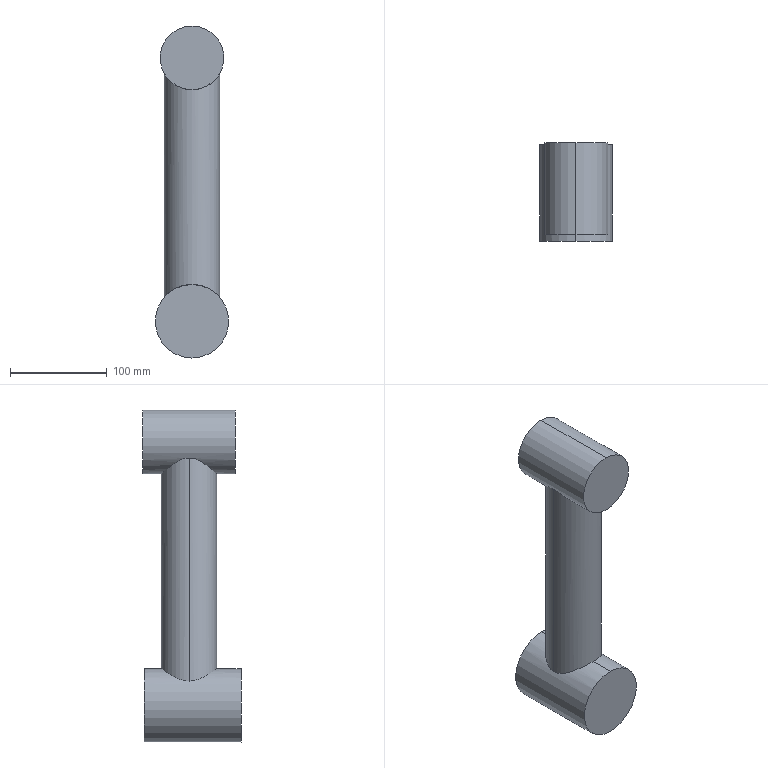Component | SolidWorks | RehabilitationChair-18-8-2 | 1 solid | 12 faces | box 75.75 x 101.12 x 342.27 mm | volume 1304986 mm3 | cylinder 6 | plane 6 | commonest cylinder face diameters 75.746 x2 65.746 x2 57.165 x2
STEP:
#1=COLOUR_RGB('',0.7922,0.8196,0.9333);
#2=FILL_AREA_STYLE_COLOUR('',#1);
#3=FILL_AREA_STYLE('',(#2));
#4=SURFACE_STYLE_FILL_AREA(#3);
#5=SURFACE_SIDE_STYLE('',(#4));
#6=SURFACE_STYLE_USAGE(.BOTH.,#5);
#7=PRESENTATION_STYLE_ASSIGNMENT((#6));
#8=CARTESIAN_POINT('',(-6.121,12.801,6.194));
#9=VERTEX_POINT('',#8);
#10=CARTESIAN_POINT('',(-6.121,12.801,3.212));
#11=VERTEX_POINT('',#10);
#12=CARTESIAN_POINT('',(-6.121,12.801,4.703));
#13=DIRECTION('',(-0.00000124,-1.,-0.));
#14=DIRECTION('',(-0.00000052,0.,1.));
#15=AXIS2_PLACEMENT_3D('',#12,#13,#14);
#16=CIRCLE('',#15,1.491);
#17=EDGE_CURVE('',#9,#11,#16,.T.);
#18=ORIENTED_EDGE('',*,*,#17,.F.);
#19=CARTESIAN_POINT('',(-6.121,13.786,6.194));
#20=VERTEX_POINT('',#19);
#21=CARTESIAN_POINT('',(-6.121,12.801,6.194));
#22=DIRECTION('',(0.00000124,1.,0.));
#23=VECTOR('',#22,39.37);
#24=LINE('',#21,#23);
#25=EDGE_CURVE('',#9,#20,#24,.T.);
#26=ORIENTED_EDGE('',*,*,#25,.T.);
#27=CARTESIAN_POINT('',(-7.246,14.911,5.682));
#28=VERTEX_POINT('',#27);
#29=CARTESIAN_POINT('',(-7.246,14.911,5.682));
#30=CARTESIAN_POINT('',(-7.246,14.833,5.682));
#31=CARTESIAN_POINT('',(-7.238,14.757,5.691));
#32=CARTESIAN_POINT('',(-7.219,14.664,5.712));
#33=CARTESIAN_POINT('',(-7.215,14.646,5.717));
#34=CARTESIAN_POINT('',(-7.205,14.61,5.727));
#35=CARTESIAN_POINT('',(-7.2,14.592,5.732));
#36=CARTESIAN_POINT('',(-7.183,14.539,5.749));
#37=CARTESIAN_POINT('',(-7.171,14.504,5.762));
#38=CARTESIAN_POINT('',(-7.128,14.405,5.803));
#39=CARTESIAN_POINT('',(-7.094,14.342,5.834));
#40=CARTESIAN_POINT('',(-7.015,14.224,5.897));
#41=CARTESIAN_POINT('',(-6.971,14.17,5.93));
#42=CARTESIAN_POINT('',(-6.896,14.095,5.977));
#43=CARTESIAN_POINT('',(-6.87,14.071,5.993));
#44=CARTESIAN_POINT('',(-6.829,14.037,6.015));
#45=CARTESIAN_POINT('',(-6.815,14.025,6.023));
#46=CARTESIAN_POINT('',(-6.787,14.004,6.038));
#47=CARTESIAN_POINT('',(-6.772,13.993,6.045));
#48=CARTESIAN_POINT('',(-6.698,13.942,6.08));
#49=CARTESIAN_POINT('',(-6.634,13.907,6.105));
#50=CARTESIAN_POINT('',(-6.531,13.863,6.137));
#51=CARTESIAN_POINT('',(-6.496,13.849,6.147));
#52=CARTESIAN_POINT('',(-6.424,13.827,6.164));
#53=CARTESIAN_POINT('',(-6.387,13.817,6.171));
#54=CARTESIAN_POINT('',(-6.313,13.802,6.182));
#55=CARTESIAN_POINT('',(-6.275,13.796,6.187));
#56=CARTESIAN_POINT('',(-6.218,13.79,6.191));
#57=CARTESIAN_POINT('',(-6.199,13.788,6.192));
#58=CARTESIAN_POINT('',(-6.16,13.786,6.194));
#59=CARTESIAN_POINT('',(-6.14,13.786,6.194));
#60=CARTESIAN_POINT('',(-6.121,13.786,6.194));
#61=B_SPLINE_CURVE_WITH_KNOTS('',3,(#29,#30,#31,#32,#33,#34,#35,#36,#37,#38,#39,#40,#41,#42,#43,#44,#45,#46,#47,#48,#49,#50,#51,#52,#53,#54,#55,#56,#57,#58,#59,#60),.UNSPECIFIED.,.F.,.F.,(4,2,2,2,2,2,2,2,2,2,2,2,2,2,2,4),(0.,0.005855,0.007319,0.008782,0.01171,0.01756,0.02342,0.02635,0.02781,0.02927,0.03513,0.03806,0.04098,0.04391,0.04538,0.04684),.UNSPECIFIED.);
#62=EDGE_CURVE('',#28,#20,#61,.T.);
#63=ORIENTED_EDGE('',*,*,#62,.F.);
#64=CARTESIAN_POINT('',(-6.121,16.036,6.194));
#65=VERTEX_POINT('',#64);
#66=CARTESIAN_POINT('',(-6.121,16.036,6.194));
#67=CARTESIAN_POINT('',(-6.199,16.036,6.194));
#68=CARTESIAN_POINT('',(-6.275,16.028,6.188));
#69=CARTESIAN_POINT('',(-6.387,16.005,6.171));
#70=CARTESIAN_POINT('',(-6.424,15.995,6.164));
#71=CARTESIAN_POINT('',(-6.496,15.972,6.147));
#72=CARTESIAN_POINT('',(-6.531,15.959,6.137));
#73=CARTESIAN_POINT('',(-6.599,15.93,6.116));
#74=CARTESIAN_POINT('',(-6.632,15.914,6.104));
#75=CARTESIAN_POINT('',(-6.681,15.887,6.085));
#76=CARTESIAN_POINT('',(-6.697,15.878,6.079));
#77=CARTESIAN_POINT('',(-6.728,15.859,6.065));
#78=CARTESIAN_POINT('',(-6.743,15.849,6.059));
#79=CARTESIAN_POINT('',(-6.817,15.798,6.023));
#80=CARTESIAN_POINT('',(-6.871,15.753,5.993));
#81=CARTESIAN_POINT('',(-6.933,15.69,5.953));
#82=CARTESIAN_POINT('',(-6.946,15.677,5.945));
#83=CARTESIAN_POINT('',(-6.969,15.65,5.929));
#84=CARTESIAN_POINT('',(-6.981,15.637,5.921));
#85=CARTESIAN_POINT('',(-7.014,15.596,5.897));
#86=CARTESIAN_POINT('',(-7.035,15.568,5.881));
#87=CARTESIAN_POINT('',(-7.074,15.51,5.85));
#88=CARTESIAN_POINT('',(-7.092,15.48,5.835));
#89=CARTESIAN_POINT('',(-7.118,15.433,5.812));
#90=CARTESIAN_POINT('',(-7.126,15.417,5.805));
#91=CARTESIAN_POINT('',(-7.142,15.385,5.79));
#92=CARTESIAN_POINT('',(-7.149,15.368,5.783));
#93=CARTESIAN_POINT('',(-7.185,15.285,5.749));
#94=CARTESIAN_POINT('',(-7.207,15.215,5.725));
#95=CARTESIAN_POINT('',(-7.23,15.104,5.7));
#96=CARTESIAN_POINT('',(-7.236,15.065,5.693));
#97=CARTESIAN_POINT('',(-7.244,14.989,5.684));
#98=CARTESIAN_POINT('',(-7.246,14.95,5.682));
#99=CARTESIAN_POINT('',(-7.246,14.911,5.682));
#100=B_SPLINE_CURVE_WITH_KNOTS('',3,(#66,#67,#68,#69,#70,#71,#72,#73,#74,#75,#76,#77,#78,#79,#80,#81,#82,#83,#84,#85,#86,#87,#88,#89,#90,#91,#92,#93,#94,#95,#96,#97,#98,#99),.UNSPECIFIED.,.F.,.F.,(4,2,2,2,2,2,2,2,2,2,2,2,2,2,2,2,4),(0.1403,0.1462,0.1491,0.152,0.1549,0.1564,0.1578,0.1637,0.1651,0.1666,0.1695,0.1724,0.1739,0.1753,0.1811,0.1841,0.187),.UNSPECIFIED.);
#101=EDGE_CURVE('',#65,#28,#100,.T.);
#102=ORIENTED_EDGE('',*,*,#101,.F.);
#103=CARTESIAN_POINT('',(-6.121,16.738,6.194));
#104=VERTEX_POINT('',#103);
#105=CARTESIAN_POINT('',(-6.121,12.801,6.194));
#106=DIRECTION('',(0.00000124,1.,0.));
#107=VECTOR('',#106,39.37);
#108=LINE('',#105,#107);
#109=EDGE_CURVE('',#65,#104,#108,.T.);
#110=ORIENTED_EDGE('',*,*,#109,.T.);
#111=CARTESIAN_POINT('',(-6.121,16.738,3.212));
#112=VERTEX_POINT('',#111);
#113=CARTESIAN_POINT('',(-6.121,16.738,4.703));
#114=DIRECTION('',(-0.00000124,-1.,-0.));
#115=DIRECTION('',(-0.00000052,0.,1.));
#116=AXIS2_PLACEMENT_3D('',#113,#114,#115);
#117=CIRCLE('',#116,1.491);
#118=EDGE_CURVE('',#104,#112,#117,.T.);
#119=ORIENTED_EDGE('',*,*,#118,.T.);
#120=CARTESIAN_POINT('',(-6.121,12.801,3.212));
#121=DIRECTION('',(0.00000124,1.,0.));
#122=VECTOR('',#121,39.37);
#123=LINE('',#120,#122);
#124=EDGE_CURVE('',#11,#112,#123,.T.);
#125=ORIENTED_EDGE('',*,*,#124,.F.);
#126=EDGE_LOOP('',(#18,#26,#63,#102,#110,#119,#125));
#127=FACE_OUTER_BOUND('',#126,.T.);
#128=CARTESIAN_POINT('',(-6.121,12.801,4.703));
#129=DIRECTION('',(0.00000124,1.,0.));
#130=DIRECTION('',(0.00000052,-0.,-1.));
#131=AXIS2_PLACEMENT_3D('',#128,#129,#130);
#132=CYLINDRICAL_SURFACE('',#131,1.491);
#133=ADVANCED_FACE('',(#127),#132,.T.);
#134=CARTESIAN_POINT('',(-6.121,13.042,16.687));
#135=VERTEX_POINT('',#134);
#136=CARTESIAN_POINT('',(-6.121,13.042,14.099));
#137=VERTEX_POINT('',#136);
#138=CARTESIAN_POINT('',(-6.121,13.042,15.393));
#139=DIRECTION('',(-0.00000124,-1.,-0.));
#140=DIRECTION('',(-0.00000052,0.,1.));
#141=AXIS2_PLACEMENT_3D('',#138,#139,#140);
#142=CIRCLE('',#141,1.294);
#143=EDGE_CURVE('',#135,#137,#142,.T.);
#144=ORIENTED_EDGE('',*,*,#143,.F.);
#145=CARTESIAN_POINT('',(-6.121,16.782,16.687));
#146=VERTEX_POINT('',#145);
#147=CARTESIAN_POINT('',(-6.121,13.042,16.687));
#148=DIRECTION('',(0.00000124,1.,0.));
#149=VECTOR('',#148,39.37);
#150=LINE('',#147,#149);
#151=EDGE_CURVE('',#135,#146,#150,.T.);
#152=ORIENTED_EDGE('',*,*,#151,.T.);
#153=CARTESIAN_POINT('',(-6.121,16.782,14.099));
#154=VERTEX_POINT('',#153);
#155=CARTESIAN_POINT('',(-6.121,16.782,15.393));
#156=DIRECTION('',(-0.00000124,-1.,-0.));
#157=DIRECTION('',(-0.00000052,0.,1.));
#158=AXIS2_PLACEMENT_3D('',#155,#156,#157);
#159=CIRCLE('',#158,1.294);
#160=EDGE_CURVE('',#146,#154,#159,.T.);
#161=ORIENTED_EDGE('',*,*,#160,.T.);
#162=CARTESIAN_POINT('',(-6.121,16.036,14.099));
#163=VERTEX_POINT('',#162);
#164=CARTESIAN_POINT('',(-6.121,13.042,14.099));
#165=DIRECTION('',(0.00000124,1.,0.));
#166=VECTOR('',#165,39.37);
#167=LINE('',#164,#166);
#168=EDGE_CURVE('',#163,#154,#167,.T.);
#169=ORIENTED_EDGE('',*,*,#168,.F.);
#170=CARTESIAN_POINT('',(-7.234,15.077,14.733));
#171=VERTEX_POINT('',#170);
#172=CARTESIAN_POINT('',(-7.234,15.077,14.733));
#173=CARTESIAN_POINT('',(-7.229,15.112,14.724));
#174=CARTESIAN_POINT('',(-7.222,15.146,14.713));
#175=CARTESIAN_POINT('',(-7.206,15.212,14.687));
#176=CARTESIAN_POINT('',(-7.196,15.243,14.673));
#177=CARTESIAN_POINT('',(-7.175,15.305,14.643));
#178=CARTESIAN_POINT('',(-7.164,15.335,14.626));
#179=CARTESIAN_POINT('',(-7.138,15.394,14.592));
#180=CARTESIAN_POINT('',(-7.123,15.423,14.574));
#181=CARTESIAN_POINT('',(-7.078,15.506,14.521));
#182=CARTESIAN_POINT('',(-7.044,15.558,14.484));
#183=CARTESIAN_POINT('',(-6.966,15.656,14.412));
#184=CARTESIAN_POINT('',(-6.924,15.702,14.376));
#185=CARTESIAN_POINT('',(-6.852,15.767,14.325));
#186=CARTESIAN_POINT('',(-6.827,15.788,14.308));
#187=CARTESIAN_POINT('',(-6.775,15.827,14.276));
#188=CARTESIAN_POINT('',(-6.748,15.846,14.261));
#189=CARTESIAN_POINT('',(-6.692,15.881,14.231));
#190=CARTESIAN_POINT('',(-6.663,15.898,14.218));
#191=CARTESIAN_POINT('',(-6.618,15.921,14.198));
#192=CARTESIAN_POINT('',(-6.602,15.928,14.192));
#193=CARTESIAN_POINT('',(-6.571,15.942,14.18));
#194=CARTESIAN_POINT('',(-6.555,15.949,14.174));
#195=CARTESIAN_POINT('',(-6.474,15.982,14.146));
#196=CARTESIAN_POINT('',(-6.407,16.002,14.129));
#197=CARTESIAN_POINT('',(-6.301,16.022,14.111));
#198=CARTESIAN_POINT('',(-6.265,16.028,14.106));
#199=CARTESIAN_POINT('',(-6.193,16.035,14.1));
#200=CARTESIAN_POINT('',(-6.157,16.036,14.099));
#201=CARTESIAN_POINT('',(-6.121,16.036,14.099));
#202=B_SPLINE_CURVE_WITH_KNOTS('',3,(#172,#173,#174,#175,#176,#177,#178,#179,#180,#181,#182,#183,#184,#185,#186,#187,#188,#189,#190,#191,#192,#193,#194,#195,#196,#197,#198,#199,#200,#201),.UNSPECIFIED.,.F.,.F.,(4,2,2,2,2,2,2,2,2,2,2,2,2,2,4),(0.,0.002745,0.005491,0.008236,0.01098,0.01647,0.02196,0.02471,0.02745,0.0302,0.03157,0.03295,0.03844,0.04118,0.04393),.UNSPECIFIED.);
#203=EDGE_CURVE('',#171,#163,#202,.T.);
#204=ORIENTED_EDGE('',*,*,#203,.F.);
#205=CARTESIAN_POINT('',(-7.234,14.745,14.733));
#206=VERTEX_POINT('',#205);
#207=CARTESIAN_POINT('',(-7.234,13.042,14.733));
#208=DIRECTION('',(0.00000124,1.,0.));
#209=VECTOR('',#208,39.37);
#210=LINE('',#207,#209);
#211=EDGE_CURVE('',#206,#171,#210,.T.);
#212=ORIENTED_EDGE('',*,*,#211,.F.);
#213=CARTESIAN_POINT('',(-6.121,13.786,14.099));
#214=VERTEX_POINT('',#213);
#215=CARTESIAN_POINT('',(-6.121,13.786,14.099));
#216=CARTESIAN_POINT('',(-6.157,13.786,14.099));
#217=CARTESIAN_POINT('',(-6.193,13.787,14.1));
#218=CARTESIAN_POINT('',(-6.247,13.793,14.105));
#219=CARTESIAN_POINT('',(-6.265,13.795,14.107));
#220=CARTESIAN_POINT('',(-6.301,13.8,14.111));
#221=CARTESIAN_POINT('',(-6.319,13.803,14.114));
#222=CARTESIAN_POINT('',(-6.406,13.82,14.129));
#223=CARTESIAN_POINT('',(-6.474,13.84,14.146));
#224=CARTESIAN_POINT('',(-6.603,13.892,14.19));
#225=CARTESIAN_POINT('',(-6.663,13.923,14.216));
#226=CARTESIAN_POINT('',(-6.734,13.967,14.253));
#227=CARTESIAN_POINT('',(-6.747,13.976,14.261));
#228=CARTESIAN_POINT('',(-6.775,13.995,14.276));
#229=CARTESIAN_POINT('',(-6.788,14.005,14.284));
#230=CARTESIAN_POINT('',(-6.827,14.034,14.308));
#231=CARTESIAN_POINT('',(-6.852,14.055,14.325));
#232=CARTESIAN_POINT('',(-6.923,14.119,14.376));
#233=CARTESIAN_POINT('',(-6.965,14.165,14.411));
#234=CARTESIAN_POINT('',(-7.024,14.238,14.465));
#235=CARTESIAN_POINT('',(-7.042,14.264,14.484));
#236=CARTESIAN_POINT('',(-7.077,14.316,14.52));
#237=CARTESIAN_POINT('',(-7.093,14.343,14.538));
#238=CARTESIAN_POINT('',(-7.138,14.426,14.592));
#239=CARTESIAN_POINT('',(-7.164,14.484,14.626));
#240=CARTESIAN_POINT('',(-7.196,14.578,14.673));
#241=CARTESIAN_POINT('',(-7.206,14.61,14.687));
#242=CARTESIAN_POINT('',(-7.222,14.676,14.713));
#243=CARTESIAN_POINT('',(-7.229,14.71,14.724));
#244=CARTESIAN_POINT('',(-7.234,14.745,14.733));
#245=B_SPLINE_CURVE_WITH_KNOTS('',3,(#215,#216,#217,#218,#219,#220,#221,#222,#223,#224,#225,#226,#227,#228,#229,#230,#231,#232,#233,#234,#235,#236,#237,#238,#239,#240,#241,#242,#243,#244),.UNSPECIFIED.,.F.,.F.,(4,2,2,2,2,2,2,2,2,2,2,2,2,2,4),(0.04393,0.04667,0.04803,0.0494,0.05488,0.06036,0.06173,0.0631,0.06583,0.07131,0.07405,0.07679,0.08227,0.085,0.08774),.UNSPECIFIED.);
#246=EDGE_CURVE('',#214,#206,#245,.T.);
#247=ORIENTED_EDGE('',*,*,#246,.F.);
#248=CARTESIAN_POINT('',(-6.121,13.042,14.099));
#249=DIRECTION('',(0.00000124,1.,0.));
#250=VECTOR('',#249,39.37);
#251=LINE('',#248,#250);
#252=EDGE_CURVE('',#137,#214,#251,.T.);
#253=ORIENTED_EDGE('',*,*,#252,.F.);
#254=EDGE_LOOP('',(#144,#152,#161,#169,#204,#212,#247,#253));
#255=FACE_OUTER_BOUND('',#254,.T.);
#256=CARTESIAN_POINT('',(-6.121,13.042,15.393));
#257=DIRECTION('',(0.00000124,1.,0.));
#258=DIRECTION('',(0.00000052,-0.,-1.));
#259=AXIS2_PLACEMENT_3D('',#256,#257,#258);
#260=CYLINDRICAL_SURFACE('',#259,1.294);
#261=ADVANCED_FACE('',(#255),#260,.T.);
#262=CARTESIAN_POINT('',(-5.008,15.077,14.733));
#263=VERTEX_POINT('',#262);
#264=CARTESIAN_POINT('',(-4.996,14.911,14.733));
#265=VERTEX_POINT('',#264);
#266=CARTESIAN_POINT('',(-6.121,14.911,14.733));
#267=DIRECTION('',(0.00000052,-0.,-1.));
#268=DIRECTION('',(1.,-0.00000124,0.00000052));
#269=AXIS2_PLACEMENT_3D('',#266,#267,#268);
#270=CIRCLE('',#269,1.125);
#271=EDGE_CURVE('',#263,#265,#270,.T.);
#272=ORIENTED_EDGE('',*,*,#271,.T.);
#273=CARTESIAN_POINT('',(-4.996,14.911,5.682));
#274=VERTEX_POINT('',#273);
#275=CARTESIAN_POINT('',(-4.996,14.911,6.828));
#276=DIRECTION('',(0.00000052,-0.,-1.));
#277=VECTOR('',#276,39.37);
#278=LINE('',#275,#277);
#279=EDGE_CURVE('',#265,#274,#278,.T.);
#280=ORIENTED_EDGE('',*,*,#279,.T.);
#281=CARTESIAN_POINT('',(-4.996,14.911,5.682));
#282=CARTESIAN_POINT('',(-4.996,14.93,5.682));
#283=CARTESIAN_POINT('',(-4.996,14.95,5.682));
#284=CARTESIAN_POINT('',(-4.998,14.989,5.684));
#285=CARTESIAN_POINT('',(-5.,15.008,5.686));
#286=CARTESIAN_POINT('',(-5.006,15.066,5.693));
#287=CARTESIAN_POINT('',(-5.011,15.103,5.7));
#288=CARTESIAN_POINT('',(-5.023,15.159,5.712));
#289=CARTESIAN_POINT('',(-5.027,15.177,5.717));
#290=CARTESIAN_POINT('',(-5.037,15.213,5.727));
#291=CARTESIAN_POINT('',(-5.042,15.231,5.732));
#292=CARTESIAN_POINT('',(-5.059,15.284,5.75));
#293=CARTESIAN_POINT('',(-5.071,15.319,5.763));
#294=CARTESIAN_POINT('',(-5.114,15.418,5.803));
#295=CARTESIAN_POINT('',(-5.148,15.48,5.834));
#296=CARTESIAN_POINT('',(-5.207,15.569,5.882));
#297=CARTESIAN_POINT('',(-5.228,15.597,5.898));
#298=CARTESIAN_POINT('',(-5.273,15.651,5.93));
#299=CARTESIAN_POINT('',(-5.296,15.677,5.946));
#300=CARTESIAN_POINT('',(-5.346,15.727,5.977));
#301=CARTESIAN_POINT('',(-5.372,15.751,5.993));
#302=CARTESIAN_POINT('',(-5.426,15.797,6.023));
#303=CARTESIAN_POINT('',(-5.455,15.819,6.038));
#304=CARTESIAN_POINT('',(-5.544,15.88,6.08));
#305=CARTESIAN_POINT('',(-5.608,15.915,6.105));
#306=CARTESIAN_POINT('',(-5.693,15.952,6.132));
#307=CARTESIAN_POINT('',(-5.711,15.959,6.137));
#308=CARTESIAN_POINT('',(-5.746,15.972,6.147));
#309=CARTESIAN_POINT('',(-5.764,15.978,6.151));
#310=CARTESIAN_POINT('',(-5.818,15.995,6.164));
#311=CARTESIAN_POINT('',(-5.855,16.005,6.171));
#312=CARTESIAN_POINT('',(-5.929,16.02,6.182));
#313=CARTESIAN_POINT('',(-5.967,16.026,6.187));
#314=CARTESIAN_POINT('',(-6.024,16.032,6.191));
#315=CARTESIAN_POINT('',(-6.043,16.034,6.192));
#316=CARTESIAN_POINT('',(-6.082,16.036,6.194));
#317=CARTESIAN_POINT('',(-6.101,16.036,6.194));
#318=CARTESIAN_POINT('',(-6.121,16.036,6.194));
#319=B_SPLINE_CURVE_WITH_KNOTS('',3,(#281,#282,#283,#284,#285,#286,#287,#288,#289,#290,#291,#292,#293,#294,#295,#296,#297,#298,#299,#300,#301,#302,#303,#304,#305,#306,#307,#308,#309,#310,#311,#312,#313,#314,#315,#316,#317,#318),.UNSPECIFIED.,.F.,.F.,(4,2,2,2,2,2,2,2,2,2,2,2,2,2,2,2,2,2,4),(0.09357,0.09503,0.0965,0.09942,0.1009,0.1023,0.1053,0.1111,0.114,0.1169,0.1199,0.1228,0.1286,0.1301,0.1316,0.1345,0.1374,0.1389,0.1403),.UNSPECIFIED.);
#320=EDGE_CURVE('',#274,#65,#319,.T.);
#321=ORIENTED_EDGE('',*,*,#320,.T.);
#322=ORIENTED_EDGE('',*,*,#101,.T.);
#323=CARTESIAN_POINT('',(-7.246,14.911,14.733));
#324=VERTEX_POINT('',#323);
#325=CARTESIAN_POINT('',(-7.246,14.911,6.828));
#326=DIRECTION('',(0.00000052,-0.,-1.));
#327=VECTOR('',#326,39.37);
#328=LINE('',#325,#327);
#329=EDGE_CURVE('',#324,#28,#328,.T.);
#330=ORIENTED_EDGE('',*,*,#329,.F.);
#331=CARTESIAN_POINT('',(-6.121,14.911,14.733));
#332=DIRECTION('',(0.00000052,-0.,-1.));
#333=DIRECTION('',(1.,-0.00000124,0.00000052));
#334=AXIS2_PLACEMENT_3D('',#331,#332,#333);
#335=CIRCLE('',#334,1.125);
#336=EDGE_CURVE('',#324,#171,#335,.T.);
#337=ORIENTED_EDGE('',*,*,#336,.T.);
#338=ORIENTED_EDGE('',*,*,#203,.T.);
#339=CARTESIAN_POINT('',(-6.121,16.036,14.099));
#340=CARTESIAN_POINT('',(-6.085,16.036,14.099));
#341=CARTESIAN_POINT('',(-6.049,16.035,14.1));
#342=CARTESIAN_POINT('',(-5.995,16.029,14.105));
#343=CARTESIAN_POINT('',(-5.977,16.027,14.107));
#344=CARTESIAN_POINT('',(-5.941,16.022,14.111));
#345=CARTESIAN_POINT('',(-5.923,16.019,14.114));
#346=CARTESIAN_POINT('',(-5.835,16.002,14.129));
#347=CARTESIAN_POINT('',(-5.768,15.982,14.146));
#348=CARTESIAN_POINT('',(-5.638,15.93,14.19));
#349=CARTESIAN_POINT('',(-5.578,15.899,14.216));
#350=CARTESIAN_POINT('',(-5.508,15.855,14.253));
#351=CARTESIAN_POINT('',(-5.494,15.846,14.261));
#352=CARTESIAN_POINT('',(-5.467,15.827,14.276));
#353=CARTESIAN_POINT('',(-5.454,15.817,14.284));
#354=CARTESIAN_POINT('',(-5.415,15.788,14.308));
#355=CARTESIAN_POINT('',(-5.39,15.767,14.325));
#356=CARTESIAN_POINT('',(-5.319,15.703,14.376));
#357=CARTESIAN_POINT('',(-5.276,15.657,14.411));
#358=CARTESIAN_POINT('',(-5.218,15.584,14.465));
#359=CARTESIAN_POINT('',(-5.2,15.558,14.484));
#360=CARTESIAN_POINT('',(-5.165,15.506,14.52));
#361=CARTESIAN_POINT('',(-5.149,15.479,14.538));
#362=CARTESIAN_POINT('',(-5.103,15.396,14.592));
#363=CARTESIAN_POINT('',(-5.077,15.338,14.626));
#364=CARTESIAN_POINT('',(-5.046,15.244,14.673));
#365=CARTESIAN_POINT('',(-5.036,15.212,14.687));
#366=CARTESIAN_POINT('',(-5.02,15.146,14.713));
#367=CARTESIAN_POINT('',(-5.013,15.112,14.724));
#368=CARTESIAN_POINT('',(-5.008,15.077,14.733));
#369=B_SPLINE_CURVE_WITH_KNOTS('',3,(#339,#340,#341,#342,#343,#344,#345,#346,#347,#348,#349,#350,#351,#352,#353,#354,#355,#356,#357,#358,#359,#360,#361,#362,#363,#364,#365,#366,#367,#368),.UNSPECIFIED.,.F.,.F.,(4,2,2,2,2,2,2,2,2,2,2,2,2,2,4),(0.04393,0.04667,0.04803,0.0494,0.05488,0.06036,0.06173,0.0631,0.06583,0.07131,0.07405,0.07679,0.08227,0.085,0.08774),.UNSPECIFIED.);
#370=EDGE_CURVE('',#163,#263,#369,.T.);
#371=ORIENTED_EDGE('',*,*,#370,.T.);
#372=EDGE_LOOP('',(#272,#280,#321,#322,#330,#337,#338,#371));
#373=FACE_OUTER_BOUND('',#372,.T.);
#374=CARTESIAN_POINT('',(-6.121,14.911,6.828));
#375=DIRECTION('',(0.00000052,-0.,-1.));
#376=DIRECTION('',(-1.,0.00000124,-0.00000052));
#377=AXIS2_PLACEMENT_3D('',#374,#375,#376);
#378=CYLINDRICAL_SURFACE('',#377,1.125);
#379=ADVANCED_FACE('',(#373),#378,.T.);
#380=ORIENTED_EDGE('',*,*,#279,.F.);
#381=CARTESIAN_POINT('',(-5.008,14.745,14.733));
#382=VERTEX_POINT('',#381);
#383=CARTESIAN_POINT('',(-6.121,14.911,14.733));
#384=DIRECTION('',(0.00000052,-0.,-1.));
#385=DIRECTION('',(1.,-0.00000124,0.00000052));
#386=AXIS2_PLACEMENT_3D('',#383,#384,#385);
#387=CIRCLE('',#386,1.125);
#388=EDGE_CURVE('',#265,#382,#387,.T.);
#389=ORIENTED_EDGE('',*,*,#388,.T.);
#390=CARTESIAN_POINT('',(-5.008,14.745,14.733));
#391=CARTESIAN_POINT('',(-5.013,14.71,14.724));
#392=CARTESIAN_POINT('',(-5.02,14.676,14.713));
#393=CARTESIAN_POINT('',(-5.036,14.61,14.687));
#394=CARTESIAN_POINT('',(-5.045,14.579,14.673));
#395=CARTESIAN_POINT('',(-5.066,14.517,14.643));
#396=CARTESIAN_POINT('',(-5.078,14.487,14.626));
#397=CARTESIAN_POINT('',(-5.104,14.428,14.592));
#398=CARTESIAN_POINT('',(-5.118,14.399,14.574));
#399=CARTESIAN_POINT('',(-5.164,14.316,14.521));
#400=CARTESIAN_POINT('',(-5.198,14.264,14.484));
#401=CARTESIAN_POINT('',(-5.275,14.166,14.412));
#402=CARTESIAN_POINT('',(-5.318,14.12,14.376));
#403=CARTESIAN_POINT('',(-5.39,14.055,14.325));
#404=CARTESIAN_POINT('',(-5.415,14.034,14.308));
#405=CARTESIAN_POINT('',(-5.467,13.995,14.276));
#406=CARTESIAN_POINT('',(-5.493,13.976,14.261));
#407=CARTESIAN_POINT('',(-5.549,13.941,14.231));
#408=CARTESIAN_POINT('',(-5.578,13.924,14.218));
#409=CARTESIAN_POINT('',(-5.624,13.901,14.198));
#410=CARTESIAN_POINT('',(-5.639,13.894,14.192));
#411=CARTESIAN_POINT('',(-5.671,13.88,14.18));
#412=CARTESIAN_POINT('',(-5.687,13.873,14.174));
#413=CARTESIAN_POINT('',(-5.767,13.84,14.146));
#414=CARTESIAN_POINT('',(-5.834,13.82,14.129));
#415=CARTESIAN_POINT('',(-5.94,13.8,14.111));
#416=CARTESIAN_POINT('',(-5.977,13.794,14.106));
#417=CARTESIAN_POINT('',(-6.049,13.787,14.1));
#418=CARTESIAN_POINT('',(-6.085,13.786,14.099));
#419=CARTESIAN_POINT('',(-6.121,13.786,14.099));
#420=B_SPLINE_CURVE_WITH_KNOTS('',3,(#390,#391,#392,#393,#394,#395,#396,#397,#398,#399,#400,#401,#402,#403,#404,#405,#406,#407,#408,#409,#410,#411,#412,#413,#414,#415,#416,#417,#418,#419),.UNSPECIFIED.,.F.,.F.,(4,2,2,2,2,2,2,2,2,2,2,2,2,2,4),(0.,0.002745,0.005491,0.008236,0.01098,0.01647,0.02196,0.02471,0.02745,0.0302,0.03157,0.03295,0.03844,0.04118,0.04393),.UNSPECIFIED.);
#421=EDGE_CURVE('',#382,#214,#420,.T.);
#422=ORIENTED_EDGE('',*,*,#421,.T.);
#423=ORIENTED_EDGE('',*,*,#246,.T.);
#424=CARTESIAN_POINT('',(-6.121,14.911,14.733));
#425=DIRECTION('',(0.00000052,-0.,-1.));
#426=DIRECTION('',(1.,-0.00000124,0.00000052));
#427=AXIS2_PLACEMENT_3D('',#424,#425,#426);
#428=CIRCLE('',#427,1.125);
#429=EDGE_CURVE('',#206,#324,#428,.T.);
#430=ORIENTED_EDGE('',*,*,#429,.T.);
#431=ORIENTED_EDGE('',*,*,#329,.T.);
#432=ORIENTED_EDGE('',*,*,#62,.T.);
#433=CARTESIAN_POINT('',(-6.121,13.786,6.194));
#434=CARTESIAN_POINT('',(-6.043,13.786,6.194));
#435=CARTESIAN_POINT('',(-5.967,13.794,6.188));
#436=CARTESIAN_POINT('',(-5.855,13.817,6.171));
#437=CARTESIAN_POINT('',(-5.817,13.827,6.164));
#438=CARTESIAN_POINT('',(-5.745,13.85,6.147));
#439=CARTESIAN_POINT('',(-5.71,13.863,6.137));
#440=CARTESIAN_POINT('',(-5.642,13.892,6.116));
#441=CARTESIAN_POINT('',(-5.609,13.908,6.104));
#442=CARTESIAN_POINT('',(-5.561,13.935,6.085));
#443=CARTESIAN_POINT('',(-5.545,13.944,6.079));
#444=CARTESIAN_POINT('',(-5.514,13.963,6.065));
#445=CARTESIAN_POINT('',(-5.499,13.973,6.058));
#446=CARTESIAN_POINT('',(-5.424,14.024,6.023));
#447=CARTESIAN_POINT('',(-5.37,14.07,5.993));
#448=CARTESIAN_POINT('',(-5.308,14.133,5.953));
#449=CARTESIAN_POINT('',(-5.296,14.146,5.945));
#450=CARTESIAN_POINT('',(-5.272,14.172,5.929));
#451=CARTESIAN_POINT('',(-5.261,14.185,5.921));
#452=CARTESIAN_POINT('',(-5.227,14.226,5.897));
#453=CARTESIAN_POINT('',(-5.206,14.254,5.881));
#454=CARTESIAN_POINT('',(-5.167,14.313,5.85));
#455=CARTESIAN_POINT('',(-5.149,14.343,5.834));
#456=CARTESIAN_POINT('',(-5.123,14.389,5.812));
#457=CARTESIAN_POINT('',(-5.115,14.405,5.804));
#458=CARTESIAN_POINT('',(-5.1,14.438,5.79));
#459=CARTESIAN_POINT('',(-5.092,14.454,5.783));
#460=CARTESIAN_POINT('',(-5.057,14.538,5.748));
#461=CARTESIAN_POINT('',(-5.034,14.608,5.725));
#462=CARTESIAN_POINT('',(-5.015,14.701,5.704));
#463=CARTESIAN_POINT('',(-5.012,14.72,5.7));
#464=CARTESIAN_POINT('',(-5.006,14.758,5.693));
#465=CARTESIAN_POINT('',(-5.003,14.777,5.691));
#466=CARTESIAN_POINT('',(-4.997,14.834,5.684));
#467=CARTESIAN_POINT('',(-4.996,14.872,5.682));
#468=CARTESIAN_POINT('',(-4.996,14.911,5.682));
#469=B_SPLINE_CURVE_WITH_KNOTS('',3,(#433,#434,#435,#436,#437,#438,#439,#440,#441,#442,#443,#444,#445,#446,#447,#448,#449,#450,#451,#452,#453,#454,#455,#456,#457,#458,#459,#460,#461,#462,#463,#464,#465,#466,#467,#468),.UNSPECIFIED.,.F.,.F.,(4,2,2,2,2,2,2,2,2,2,2,2,2,2,2,2,2,4),(0.04684,0.05268,0.0556,0.05852,0.06144,0.0629,0.06436,0.07021,0.07167,0.07313,0.07605,0.07897,0.08043,0.08189,0.08773,0.08919,0.09065,0.09357),.UNSPECIFIED.);
#470=EDGE_CURVE('',#20,#274,#469,.T.);
#471=ORIENTED_EDGE('',*,*,#470,.T.);
#472=EDGE_LOOP('',(#380,#389,#422,#423,#430,#431,#432,#471));
#473=FACE_OUTER_BOUND('',#472,.T.);
#474=CARTESIAN_POINT('',(-6.121,14.911,6.828));
#475=DIRECTION('',(0.00000052,-0.,-1.));
#476=DIRECTION('',(-1.,0.00000124,-0.00000052));
#477=AXIS2_PLACEMENT_3D('',#474,#475,#476);
#478=CYLINDRICAL_SURFACE('',#477,1.125);
#479=ADVANCED_FACE('',(#473),#478,.T.);
#480=ORIENTED_EDGE('',*,*,#271,.F.);
#481=CARTESIAN_POINT('',(-5.008,13.042,14.733));
#482=DIRECTION('',(-0.00000124,-1.,-0.));
#483=VECTOR('',#482,39.37);
#484=LINE('',#481,#483);
#485=EDGE_CURVE('',#263,#382,#484,.T.);
#486=ORIENTED_EDGE('',*,*,#485,.T.);
#487=ORIENTED_EDGE('',*,*,#388,.F.);
#488=EDGE_LOOP('',(#480,#486,#487));
#489=FACE_OUTER_BOUND('',#488,.T.);
#490=CARTESIAN_POINT('',(-6.121,14.911,14.733));
#491=DIRECTION('',(-0.00000052,0.,1.));
#492=DIRECTION('',(1.,-0.00000124,0.00000052));
#493=AXIS2_PLACEMENT_3D('',#490,#491,#492);
#494=PLANE('',#493);
#495=ADVANCED_FACE('',(#489),#494,.T.);
#496=ORIENTED_EDGE('',*,*,#429,.F.);
#497=ORIENTED_EDGE('',*,*,#211,.T.);
#498=ORIENTED_EDGE('',*,*,#336,.F.);
#499=EDGE_LOOP('',(#496,#497,#498));
#500=FACE_OUTER_BOUND('',#499,.T.);
#501=CARTESIAN_POINT('',(-6.121,14.911,14.733));
#502=DIRECTION('',(-0.00000052,0.,1.));
#503=DIRECTION('',(1.,-0.00000124,0.00000052));
#504=AXIS2_PLACEMENT_3D('',#501,#502,#503);
#505=PLANE('',#504);
#506=ADVANCED_FACE('',(#500),#505,.T.);
#507=ORIENTED_EDGE('',*,*,#151,.F.);
#508=CARTESIAN_POINT('',(-6.121,13.042,15.393));
#509=DIRECTION('',(-0.00000124,-1.,-0.));
#510=DIRECTION('',(-0.00000052,0.,1.));
#511=AXIS2_PLACEMENT_3D('',#508,#509,#510);
#512=CIRCLE('',#511,1.294);
#513=EDGE_CURVE('',#137,#135,#512,.T.);
#514=ORIENTED_EDGE('',*,*,#513,.F.);
#515=ORIENTED_EDGE('',*,*,#252,.T.);
#516=ORIENTED_EDGE('',*,*,#421,.F.);
#517=ORIENTED_EDGE('',*,*,#485,.F.);
#518=ORIENTED_EDGE('',*,*,#370,.F.);
#519=ORIENTED_EDGE('',*,*,#168,.T.);
#520=CARTESIAN_POINT('',(-6.121,16.782,15.393));
#521=DIRECTION('',(-0.00000124,-1.,-0.));
#522=DIRECTION('',(-0.00000052,0.,1.));
#523=AXIS2_PLACEMENT_3D('',#520,#521,#522);
#524=CIRCLE('',#523,1.294);
#525=EDGE_CURVE('',#154,#146,#524,.T.);
#526=ORIENTED_EDGE('',*,*,#525,.T.);
#527=EDGE_LOOP('',(#507,#514,#515,#516,#517,#518,#519,#526));
#528=FACE_OUTER_BOUND('',#527,.T.);
#529=CARTESIAN_POINT('',(-6.121,13.042,15.393));
#530=DIRECTION('',(0.00000124,1.,0.));
#531=DIRECTION('',(0.00000052,-0.,-1.));
#532=AXIS2_PLACEMENT_3D('',#529,#530,#531);
#533=CYLINDRICAL_SURFACE('',#532,1.294);
#534=ADVANCED_FACE('',(#528),#533,.T.);
#535=ORIENTED_EDGE('',*,*,#513,.T.);
#536=ORIENTED_EDGE('',*,*,#143,.T.);
#537=EDGE_LOOP('',(#535,#536));
#538=FACE_OUTER_BOUND('',#537,.T.);
#539=CARTESIAN_POINT('',(-6.121,13.042,15.393));
#540=DIRECTION('',(-0.00000124,-1.,-0.));
#541=DIRECTION('',(-0.00000052,0.,1.));
#542=AXIS2_PLACEMENT_3D('',#539,#540,#541);
#543=PLANE('',#542);
#544=ADVANCED_FACE('',(#538),#543,.T.);
#545=ORIENTED_EDGE('',*,*,#525,.F.);
#546=ORIENTED_EDGE('',*,*,#160,.F.);
#547=EDGE_LOOP('',(#545,#546));
#548=FACE_OUTER_BOUND('',#547,.T.);
#549=CARTESIAN_POINT('',(-6.121,16.782,15.393));
#550=DIRECTION('',(-0.00000124,-1.,-0.));
#551=DIRECTION('',(-0.00000052,0.,1.));
#552=AXIS2_PLACEMENT_3D('',#549,#550,#551);
#553=PLANE('',#552);
#554=ADVANCED_FACE('',(#548),#553,.F.);
#555=ORIENTED_EDGE('',*,*,#25,.F.);
#556=CARTESIAN_POINT('',(-6.121,12.801,4.703));
#557=DIRECTION('',(-0.00000124,-1.,-0.));
#558=DIRECTION('',(-0.00000052,0.,1.));
#559=AXIS2_PLACEMENT_3D('',#556,#557,#558);
#560=CIRCLE('',#559,1.491);
#561=EDGE_CURVE('',#11,#9,#560,.T.);
#562=ORIENTED_EDGE('',*,*,#561,.F.);
#563=ORIENTED_EDGE('',*,*,#124,.T.);
#564=CARTESIAN_POINT('',(-6.121,16.738,4.703));
#565=DIRECTION('',(-0.00000124,-1.,-0.));
#566=DIRECTION('',(-0.00000052,0.,1.));
#567=AXIS2_PLACEMENT_3D('',#564,#565,#566);
#568=CIRCLE('',#567,1.491);
#569=EDGE_CURVE('',#112,#104,#568,.T.);
#570=ORIENTED_EDGE('',*,*,#569,.T.);
#571=ORIENTED_EDGE('',*,*,#109,.F.);
#572=ORIENTED_EDGE('',*,*,#320,.F.);
#573=ORIENTED_EDGE('',*,*,#470,.F.);
#574=EDGE_LOOP('',(#555,#562,#563,#570,#571,#572,#573));
#575=FACE_OUTER_BOUND('',#574,.T.);
#576=CARTESIAN_POINT('',(-6.121,12.801,4.703));
#577=DIRECTION('',(0.00000124,1.,0.));
#578=DIRECTION('',(0.00000052,-0.,-1.));
#579=AXIS2_PLACEMENT_3D('',#576,#577,#578);
#580=CYLINDRICAL_SURFACE('',#579,1.491);
#581=ADVANCED_FACE('',(#575),#580,.T.);
#582=ORIENTED_EDGE('',*,*,#561,.T.);
#583=ORIENTED_EDGE('',*,*,#17,.T.);
#584=EDGE_LOOP('',(#582,#583));
#585=FACE_OUTER_BOUND('',#584,.T.);
#586=CARTESIAN_POINT('',(-6.121,12.801,4.703));
#587=DIRECTION('',(-0.00000124,-1.,-0.));
#588=DIRECTION('',(-0.00000052,0.,1.));
#589=AXIS2_PLACEMENT_3D('',#586,#587,#588);
#590=PLANE('',#589);
#591=ADVANCED_FACE('',(#585),#590,.T.);
#592=ORIENTED_EDGE('',*,*,#569,.F.);
#593=ORIENTED_EDGE('',*,*,#118,.F.);
#594=EDGE_LOOP('',(#592,#593));
#595=FACE_OUTER_BOUND('',#594,.T.);
#596=CARTESIAN_POINT('',(-6.121,16.738,4.703));
#597=DIRECTION('',(-0.00000124,-1.,-0.));
#598=DIRECTION('',(-0.00000052,0.,1.));
#599=AXIS2_PLACEMENT_3D('',#596,#597,#598);
#600=PLANE('',#599);
#601=ADVANCED_FACE('',(#595),#600,.F.);
#602=CLOSED_SHELL('',(#133,#261,#379,#479,#495,#506,#534,#544,#554,#581,#591,#601));
#603=MANIFOLD_SOLID_BREP('',#602);
#604=STYLED_ITEM('',(#7),#603);
#605=PRESENTATION_LAYER_ASSIGNMENT('','',(#604));
#606=CARTESIAN_POINT('',(0.,0.,0.));
#607=DIRECTION('',(0.,0.,1.));
#608=DIRECTION('',(1.,0.,0.));
#609=AXIS2_PLACEMENT_3D('',#606,#607,#608);
#610=(LENGTH_UNIT()NAMED_UNIT(*)SI_UNIT($,.METRE.));
#611=LENGTH_MEASURE_WITH_UNIT(LENGTH_MEASURE(0.0254),#610);
#612=DIMENSIONAL_EXPONENTS(1.,0.,0.,0.,0.,0.,0.);
#613=(CONVERSION_BASED_UNIT('',#611)LENGTH_UNIT()NAMED_UNIT(#612));
#614=UNCERTAINTY_MEASURE_WITH_UNIT(LENGTH_MEASURE(0.00001),#613,'','');
#615=(NAMED_UNIT(*)PLANE_ANGLE_UNIT()SI_UNIT($,.RADIAN.));
#616=(NAMED_UNIT(*)SI_UNIT($,.STERADIAN.)SOLID_ANGLE_UNIT());
#617=(GEOMETRIC_REPRESENTATION_CONTEXT(3)GLOBAL_UNCERTAINTY_ASSIGNED_CONTEXT((#614))GLOBAL_UNIT_ASSIGNED_CONTEXT((#613,#615,#616))REPRESENTATION_CONTEXT('',''));
#618=ADVANCED_BREP_SHAPE_REPRESENTATION('',(#603,#609),#617);
#619=(LENGTH_UNIT()NAMED_UNIT(*)SI_UNIT($,.METRE.));
#620=LENGTH_MEASURE_WITH_UNIT(LENGTH_MEASURE(0.0254),#619);
#621=DIMENSIONAL_EXPONENTS(1.,0.,0.,0.,0.,0.,0.);
#622=(CONVERSION_BASED_UNIT('',#620)LENGTH_UNIT()NAMED_UNIT(#621));
#623=UNCERTAINTY_MEASURE_WITH_UNIT(LENGTH_MEASURE(0.00001),#622,'','');
#624=(NAMED_UNIT(*)PLANE_ANGLE_UNIT()SI_UNIT($,.RADIAN.));
#625=(NAMED_UNIT(*)SI_UNIT($,.STERADIAN.)SOLID_ANGLE_UNIT());
#626=(GEOMETRIC_REPRESENTATION_CONTEXT(3)GLOBAL_UNCERTAINTY_ASSIGNED_CONTEXT((#623))GLOBAL_UNIT_ASSIGNED_CONTEXT((#622,#624,#625))REPRESENTATION_CONTEXT('',''));
#627=MECHANICAL_DESIGN_GEOMETRIC_PRESENTATION_REPRESENTATION('',(#604),#626);